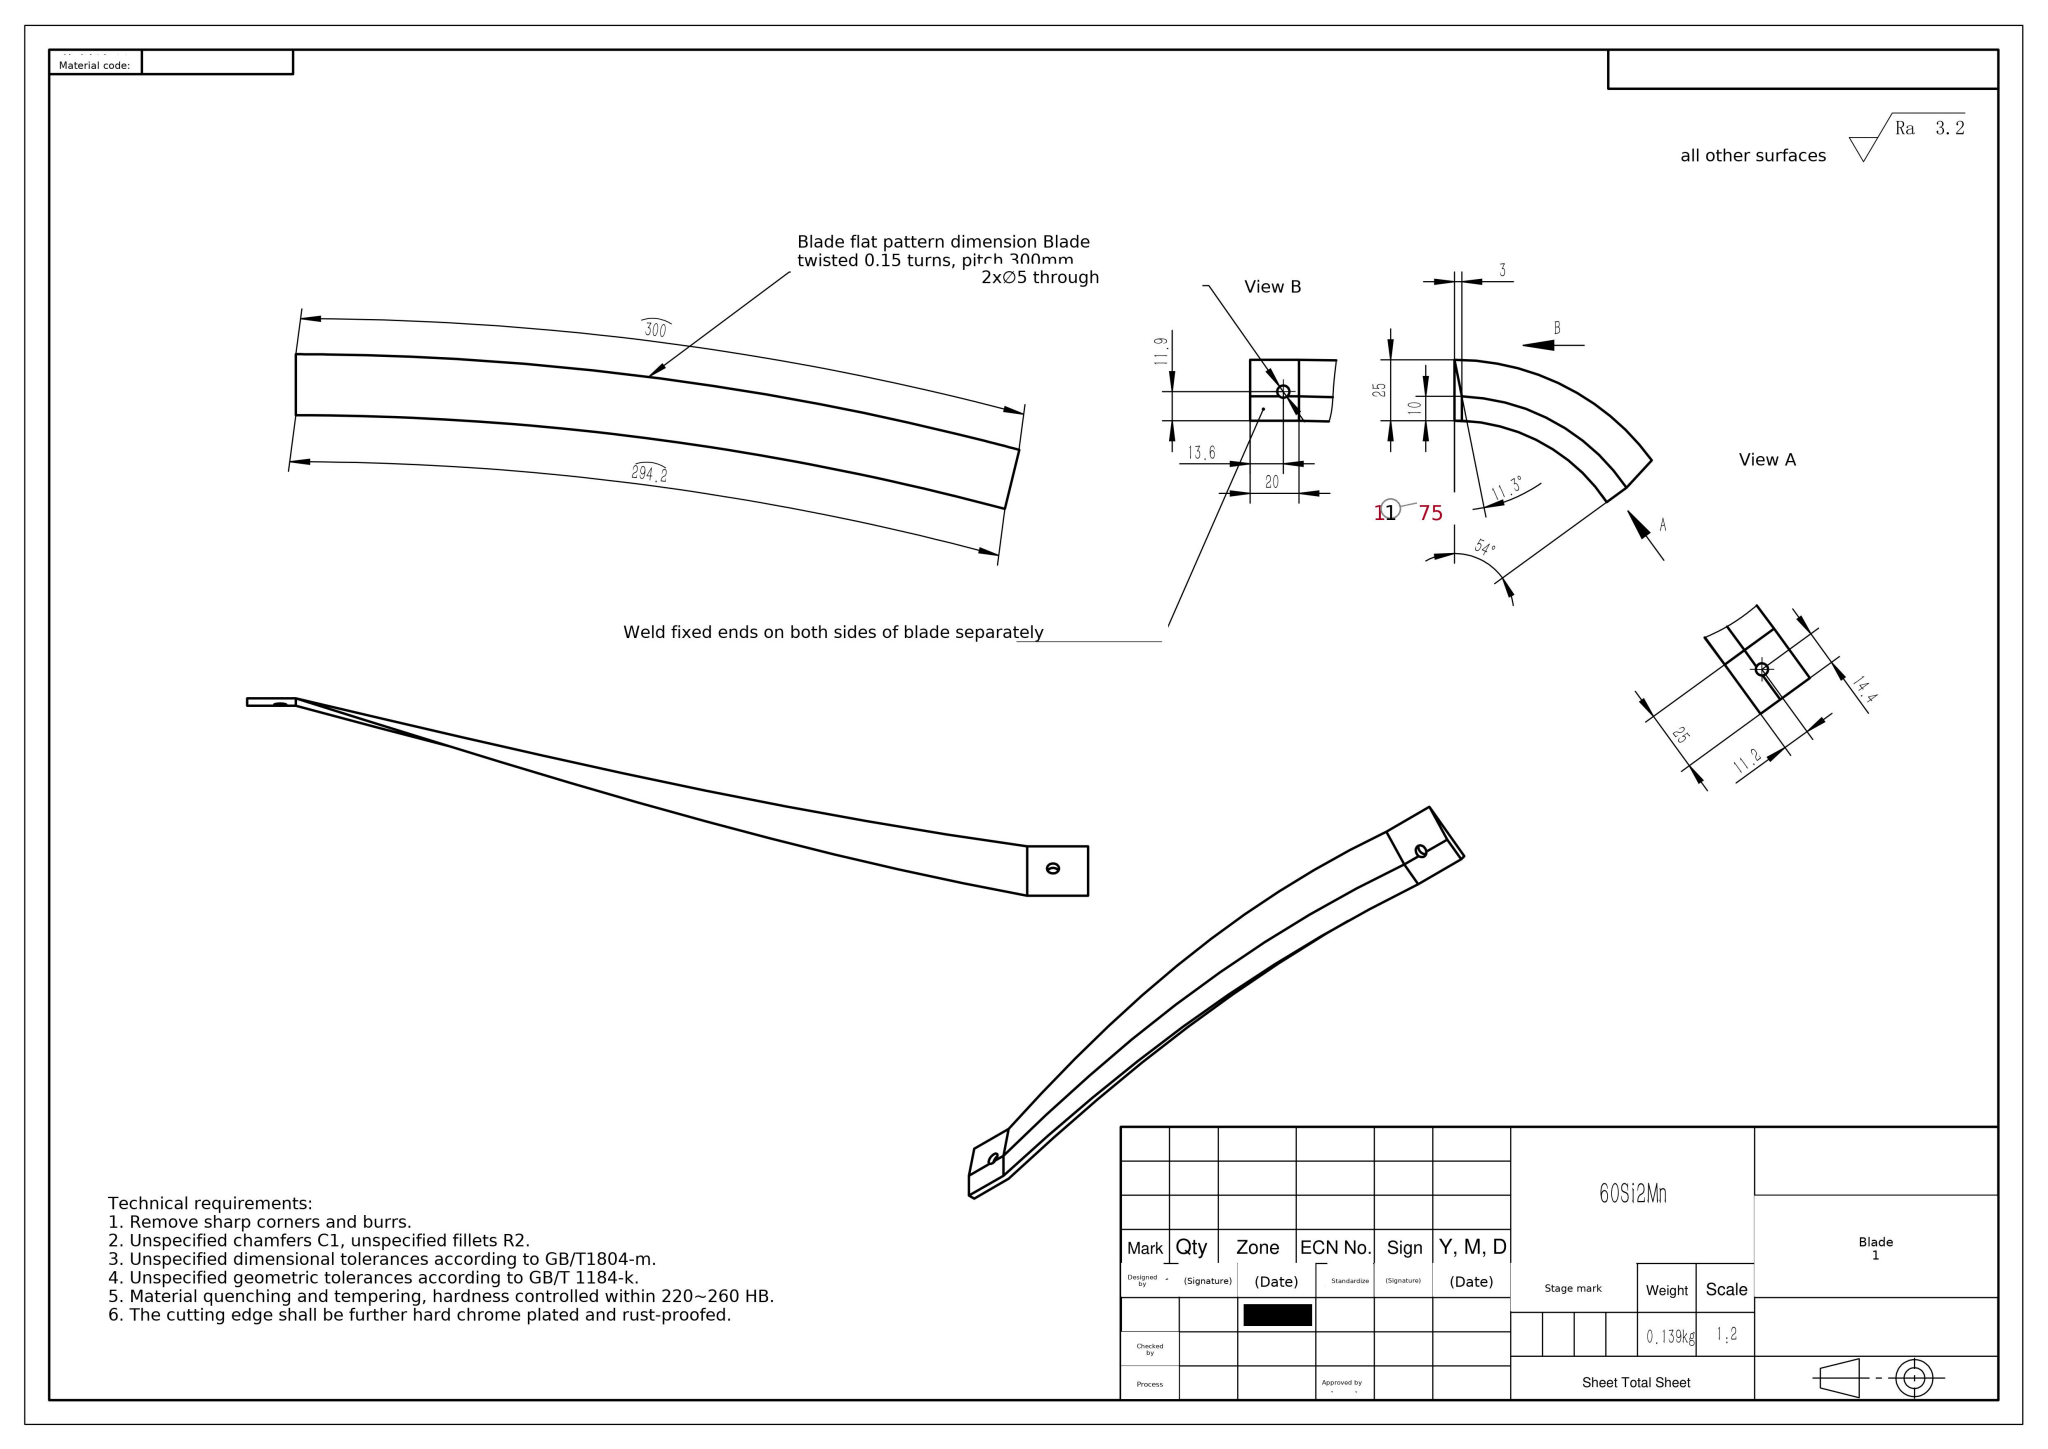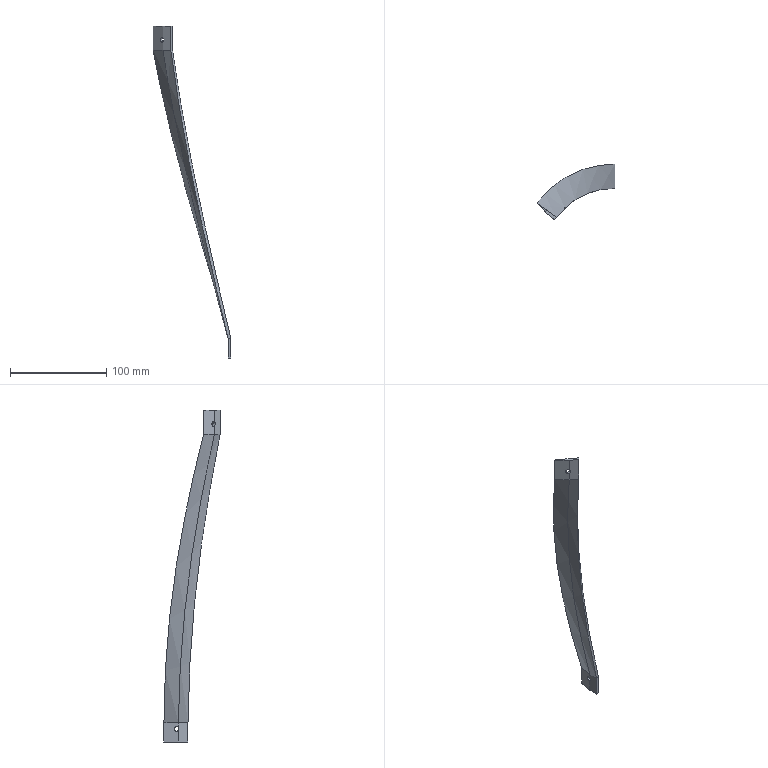Part | SolidWorks | mm | material 60Si2Mn | 1 solid | 18 faces | box 80.9 x 58.34 x 345 mm | volume 18008 mm3 | plane 10 | cylinder 4 | spline 4 | commonest cylinder face diameters 5 x4
build123d program:
from build123d import *

# Parameters (mm, degrees)
SWEEP1_PITCH             = 2000
SWEEP1_HEIGHT            = 300
SWEEP1_RADIUS            = 100
SWEEP1_START_ANGLE       = 90
BOSS_EXTRUDE1_DEPTH      = 20
BOSS_EXTRUDE2_DEPTH      = 25
F_5_0_5_DIAMETER_HOLE1_D = 5
F_5_0_5_DIAMETER_HOLE2_D = 5


with BuildPart() as part:
    # Sweep1: sweep along a helix
    with BuildLine() as sweep1_path:
        add(Helix(SWEEP1_PITCH, SWEEP1_HEIGHT, SWEEP1_RADIUS, center=(0, 0, 0), direction=(0, 0, 1), mode=Mode.PRIVATE).rotate(Axis((0, 0, 0), (0, 0, 1)), SWEEP1_START_ANGLE))
    # Sketch4 → Sweep1 (sweep)
    with BuildSketch(Plane.XY):
        Polygon((0, 100), (0, 75), (-3, 75), (-3, 85), align=None)
    sweep(path=sweep1_path.line, is_frenet=True)

    # Sketch6 → Boss-Extrude1 (add)
    with BuildSketch(Plane(origin=(0, 0, 0), x_dir=(-1, 0, 0), z_dir=(0, 0, -1))):
        Polygon((0, 75), (3, 75), (3, 85), (0, 100), align=None)
    extrude(amount=BOSS_EXTRUDE1_DEPTH)

    # Sketch7 → Boss-Extrude2 (add)
    with BuildSketch(Plane.XY.offset(300)):
        Polygon((-62.44, 41.657), (-60.676, 44.084), (-80.902, 58.779), (-70.53, 47.535), align=None)
    extrude(amount=BOSS_EXTRUDE2_DEPTH)

    # 5.0 _5_ Diameter Hole1 (through all)
    with Locations(Plane(origin=(0, 0, 0), x_dir=(0, 0, -1), z_dir=(1, 0, 0))):
        with Locations((6.423, 86.948)):
            Hole(F_5_0_5_DIAMETER_HOLE1_D / 2)

    # 5.0 _5_ Diameter Hole2 (through all)
    with Locations(Plane(origin=(0, 0, 0), x_dir=(0.809, -0.5878, 0), z_dir=(0.5878, 0.809, 0))):
        with Locations((-86.183, -310.577)):
            Hole(F_5_0_5_DIAMETER_HOLE2_D / 2)


solid = part.part